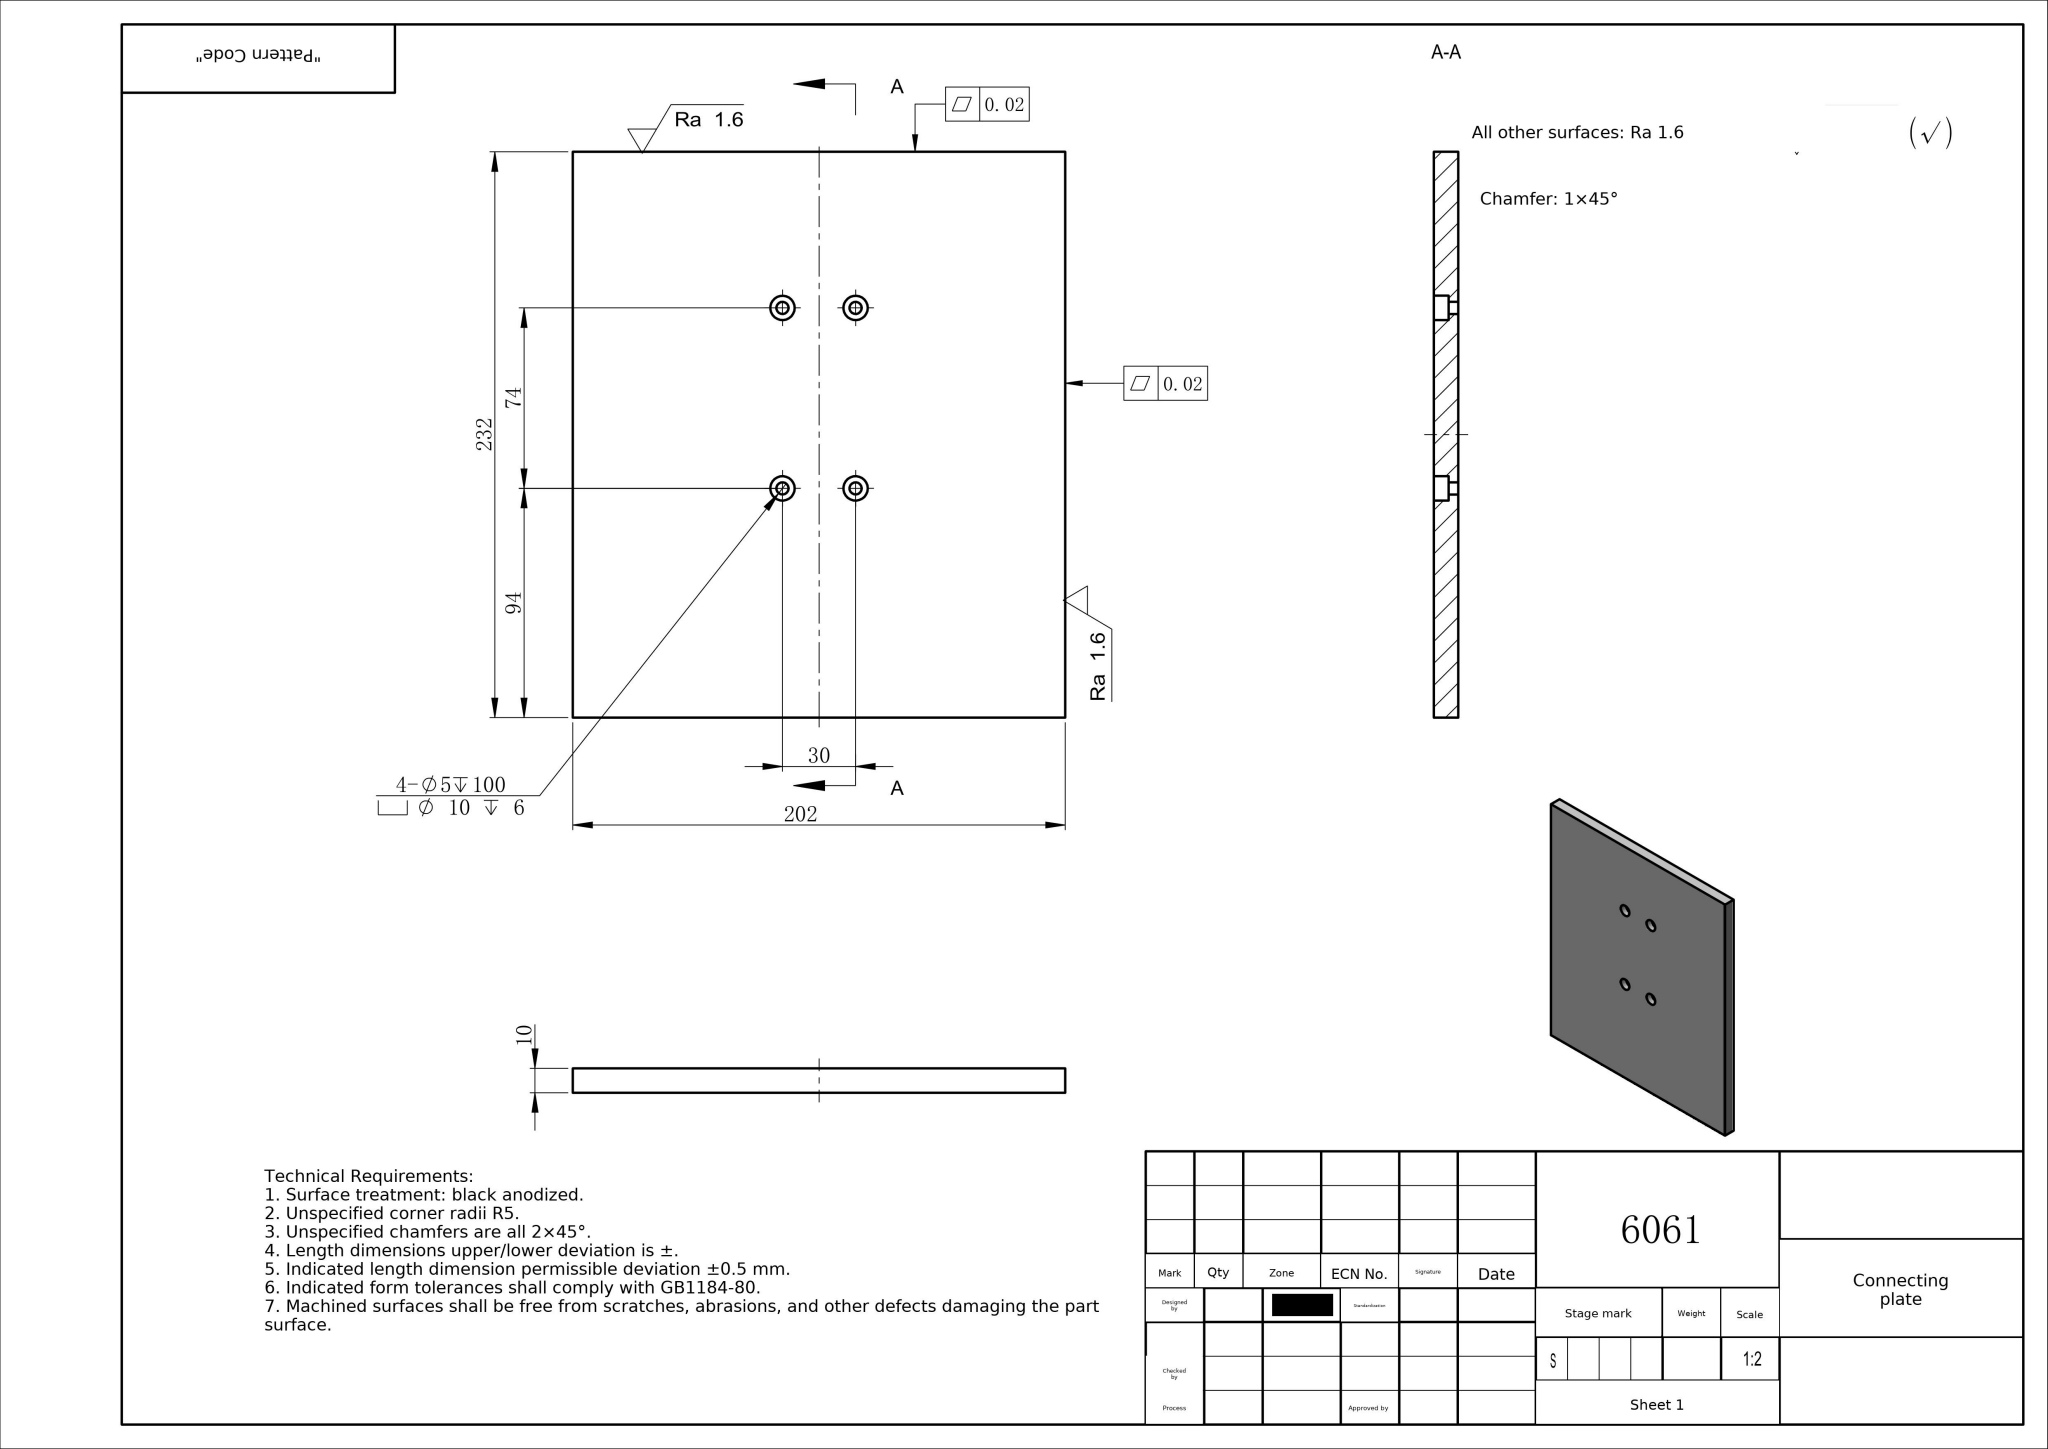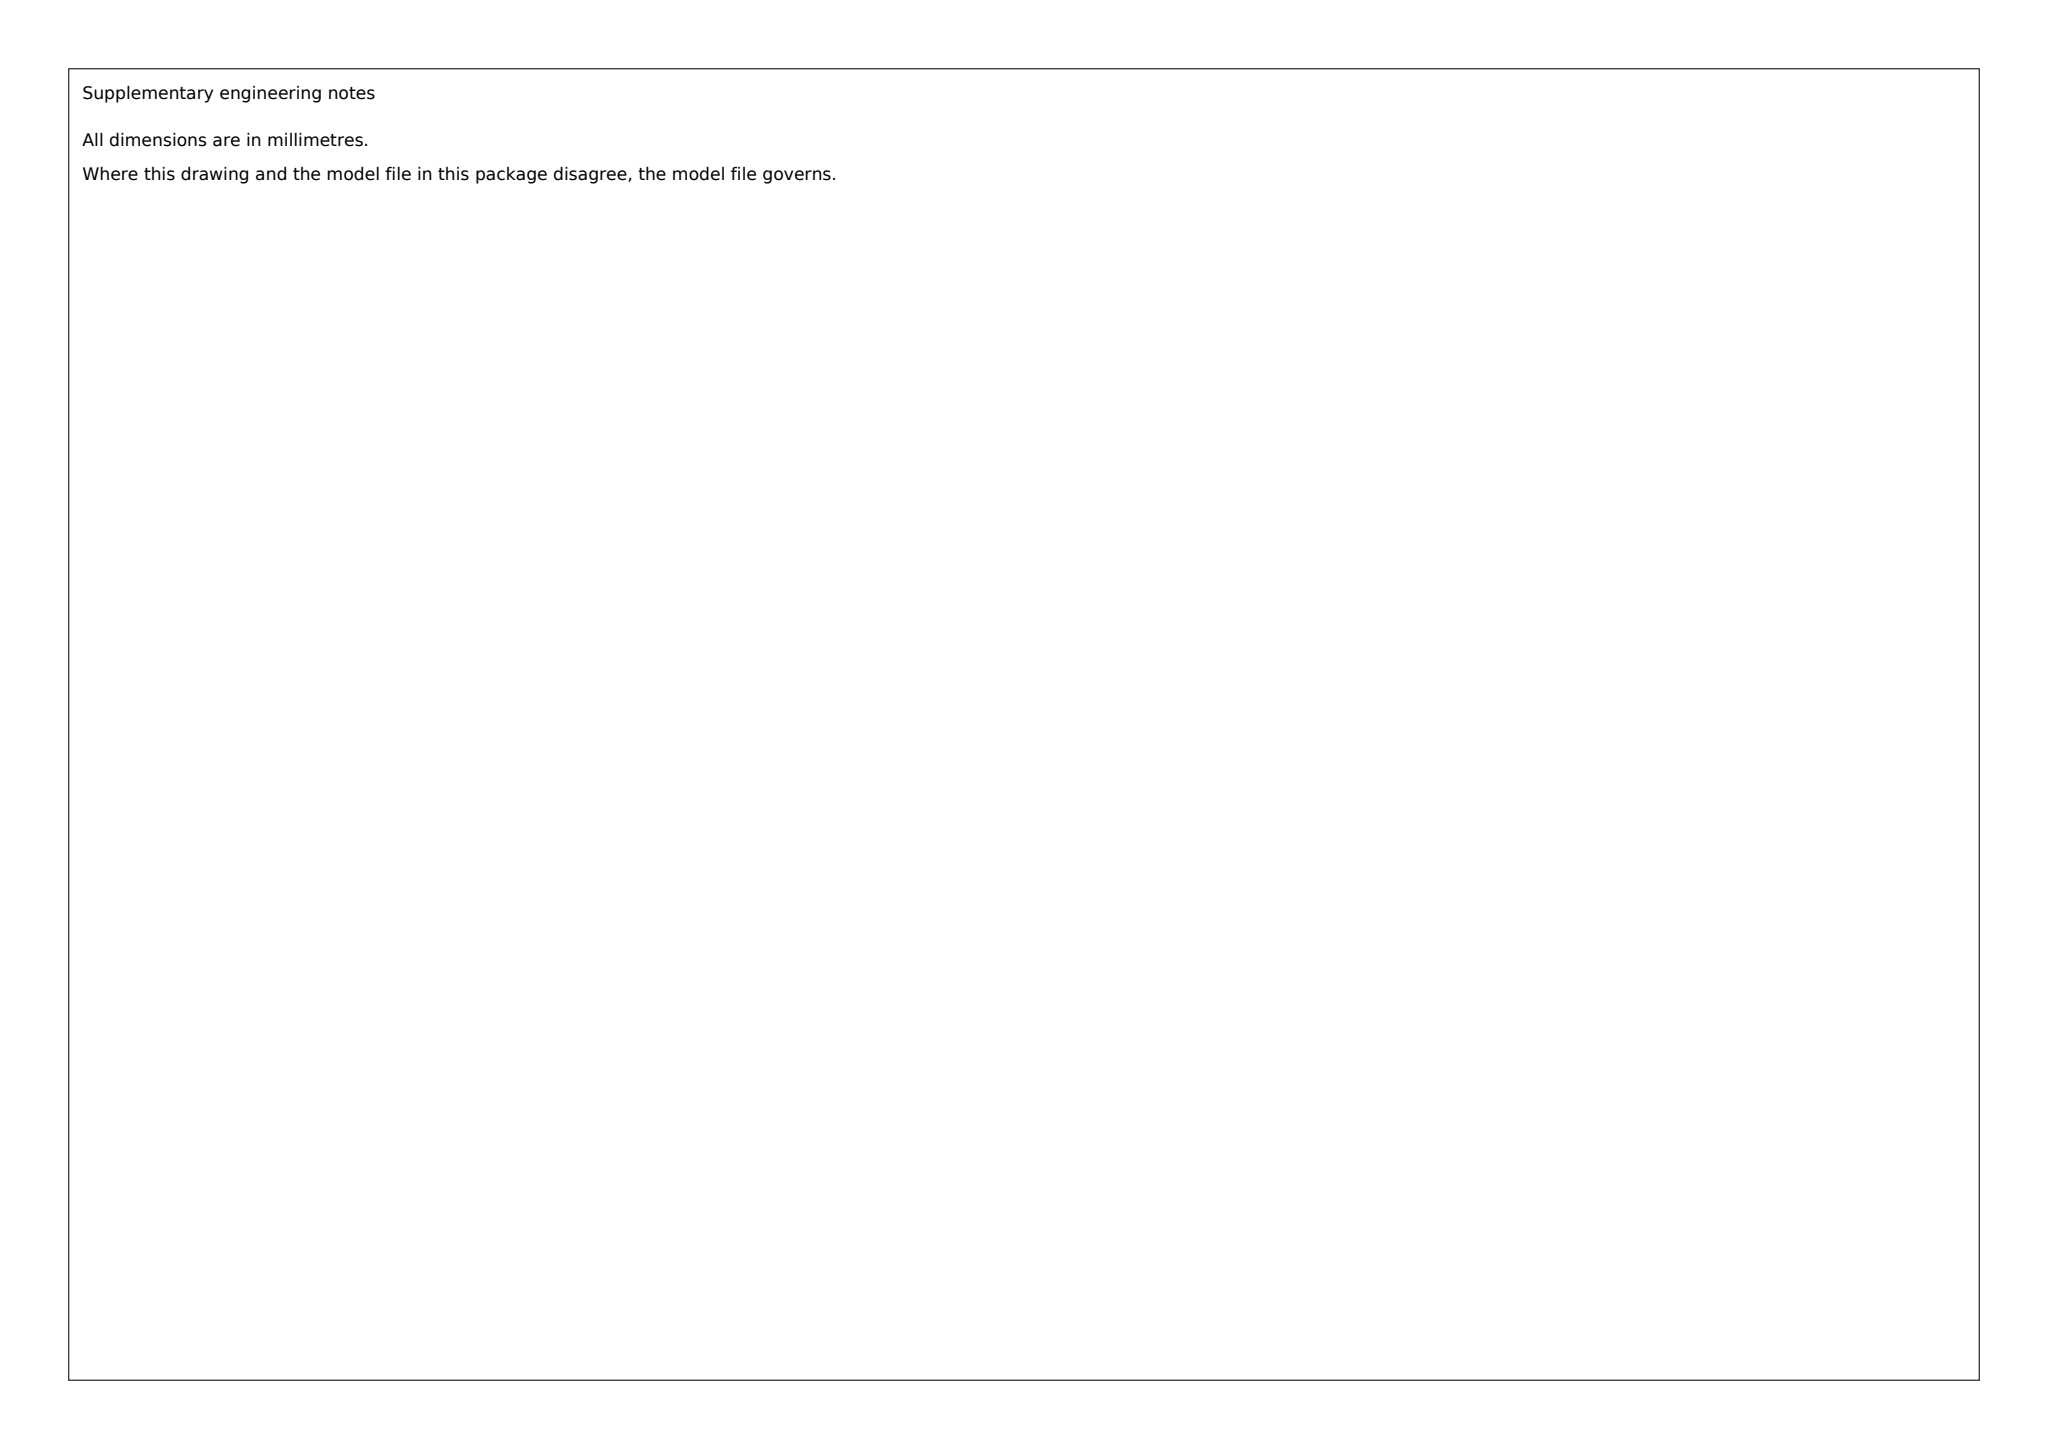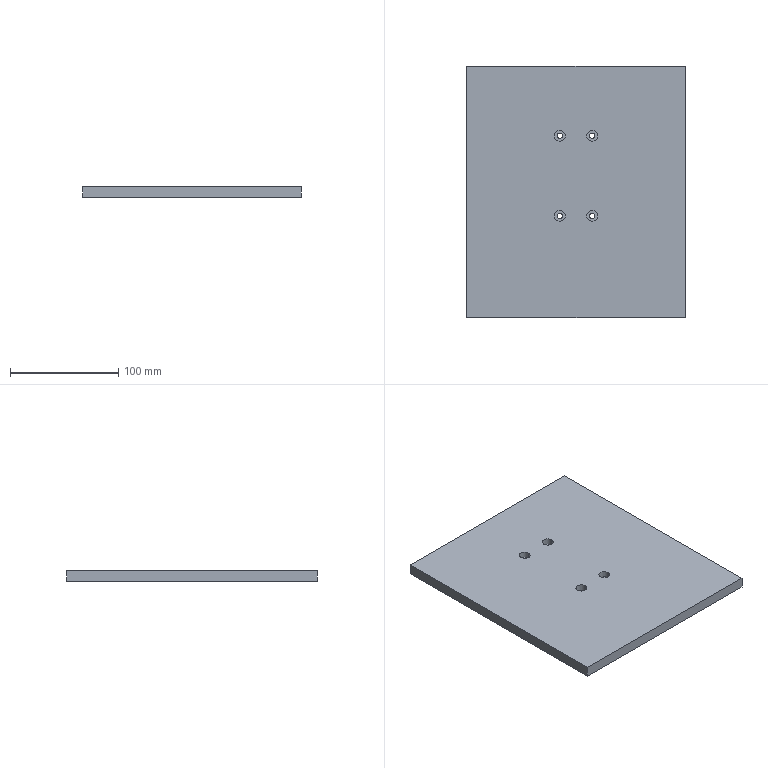Part | SolidWorks | mm | 1 solid | 26 faces | box 202 x 232 x 10 mm | volume 466441 mm3 | cylinder 16 | plane 10 | commonest cylinder face diameters 10 x8 5 x8
build123d program:
from build123d import *

# Parameters (mm, degrees)
SKETCH1_W           = 202
SKETCH1_H           = 202
BOSS_EXTRUDE1_DEPTH = 10
HOLE1_D             = 5
HOLE1_DEPTH         = 100
HOLE1_CBORE_D       = 10
HOLE1_CBORE_DEPTH   = 6
MOVE_FACE1_BY       = 30


with BuildPart() as part:
    # Sketch1 → Boss-Extrude1 (new body)
    with BuildSketch(Plane.XY):
        with Locations((-50, 0)):
            Rectangle(SKETCH1_W, SKETCH1_H)
    extrude(amount=BOSS_EXTRUDE1_DEPTH)

    # Hole1
    with Locations(Plane.XY.offset(10)):
        with Locations((-65, -37), (-65, 37), (-35, 37), (-35, -37)):
            CounterBoreHole(HOLE1_D / 2, HOLE1_CBORE_D / 2, HOLE1_CBORE_DEPTH, depth=HOLE1_DEPTH)

    # Move Face1: a face moved outward by 30.0
    extrude(part.faces().sort_by_distance((-50, -101, 5))[0], amount=MOVE_FACE1_BY, dir=(0, -1, 0))


solid = part.part
STEP:
#1=CARTESIAN_POINT('',(-70.,37.,4.));
#2=VERTEX_POINT('',#1);
#3=CARTESIAN_POINT('',(-60.,37.,4.));
#4=VERTEX_POINT('',#3);
#5=CARTESIAN_POINT('',(-65.,37.,4.));
#6=DIRECTION('',(-0.,0.,1.));
#7=DIRECTION('',(1.,0.,0.));
#8=AXIS2_PLACEMENT_3D('',#5,#6,#7);
#9=CIRCLE('',#8,5.);
#10=EDGE_CURVE('',#2,#4,#9,.T.);
#11=ORIENTED_EDGE('',*,*,#10,.F.);
#12=CARTESIAN_POINT('',(-70.,37.,10.));
#13=VERTEX_POINT('',#12);
#14=CARTESIAN_POINT('',(-70.,37.,10.));
#15=DIRECTION('',(-0.,0.,1.));
#16=VECTOR('',#15,1000.);
#17=LINE('',#14,#16);
#18=EDGE_CURVE('',#2,#13,#17,.T.);
#19=ORIENTED_EDGE('',*,*,#18,.T.);
#20=CARTESIAN_POINT('',(-60.,37.,10.));
#21=VERTEX_POINT('',#20);
#22=CARTESIAN_POINT('',(-65.,37.,10.));
#23=DIRECTION('',(-0.,0.,1.));
#24=DIRECTION('',(1.,0.,0.));
#25=AXIS2_PLACEMENT_3D('',#22,#23,#24);
#26=CIRCLE('',#25,5.);
#27=EDGE_CURVE('',#13,#21,#26,.T.);
#28=ORIENTED_EDGE('',*,*,#27,.T.);
#29=CARTESIAN_POINT('',(-60.,37.,10.));
#30=DIRECTION('',(-0.,0.,1.));
#31=VECTOR('',#30,1000.);
#32=LINE('',#29,#31);
#33=EDGE_CURVE('',#4,#21,#32,.T.);
#34=ORIENTED_EDGE('',*,*,#33,.F.);
#35=EDGE_LOOP('',(#11,#19,#28,#34));
#36=FACE_OUTER_BOUND('',#35,.T.);
#37=CARTESIAN_POINT('',(-65.,37.,10.));
#38=DIRECTION('',(-0.,0.,1.));
#39=DIRECTION('',(1.,0.,0.));
#40=AXIS2_PLACEMENT_3D('',#37,#38,#39);
#41=CYLINDRICAL_SURFACE('',#40,5.);
#42=ADVANCED_FACE('',(#36),#41,.F.);
#43=CARTESIAN_POINT('',(-67.5,37.,0.));
#44=VERTEX_POINT('',#43);
#45=CARTESIAN_POINT('',(-62.5,37.,0.));
#46=VERTEX_POINT('',#45);
#47=CARTESIAN_POINT('',(-65.,37.,0.));
#48=DIRECTION('',(-0.,0.,1.));
#49=DIRECTION('',(1.,0.,0.));
#50=AXIS2_PLACEMENT_3D('',#47,#48,#49);
#51=CIRCLE('',#50,2.5);
#52=EDGE_CURVE('',#44,#46,#51,.T.);
#53=ORIENTED_EDGE('',*,*,#52,.F.);
#54=CARTESIAN_POINT('',(-67.5,37.,4.));
#55=VERTEX_POINT('',#54);
#56=CARTESIAN_POINT('',(-67.5,37.,10.));
#57=DIRECTION('',(-0.,0.,1.));
#58=VECTOR('',#57,1000.);
#59=LINE('',#56,#58);
#60=EDGE_CURVE('',#44,#55,#59,.T.);
#61=ORIENTED_EDGE('',*,*,#60,.T.);
#62=CARTESIAN_POINT('',(-62.5,37.,4.));
#63=VERTEX_POINT('',#62);
#64=CARTESIAN_POINT('',(-65.,37.,4.));
#65=DIRECTION('',(-0.,0.,1.));
#66=DIRECTION('',(1.,0.,0.));
#67=AXIS2_PLACEMENT_3D('',#64,#65,#66);
#68=CIRCLE('',#67,2.5);
#69=EDGE_CURVE('',#55,#63,#68,.T.);
#70=ORIENTED_EDGE('',*,*,#69,.T.);
#71=CARTESIAN_POINT('',(-62.5,37.,10.));
#72=DIRECTION('',(-0.,0.,1.));
#73=VECTOR('',#72,1000.);
#74=LINE('',#71,#73);
#75=EDGE_CURVE('',#46,#63,#74,.T.);
#76=ORIENTED_EDGE('',*,*,#75,.F.);
#77=EDGE_LOOP('',(#53,#61,#70,#76));
#78=FACE_OUTER_BOUND('',#77,.T.);
#79=CARTESIAN_POINT('',(-65.,37.,10.));
#80=DIRECTION('',(-0.,0.,1.));
#81=DIRECTION('',(1.,0.,0.));
#82=AXIS2_PLACEMENT_3D('',#79,#80,#81);
#83=CYLINDRICAL_SURFACE('',#82,2.5);
#84=ADVANCED_FACE('',(#78),#83,.F.);
#85=CARTESIAN_POINT('',(-40.,37.,4.));
#86=VERTEX_POINT('',#85);
#87=CARTESIAN_POINT('',(-30.,37.,4.));
#88=VERTEX_POINT('',#87);
#89=CARTESIAN_POINT('',(-35.,37.,4.));
#90=DIRECTION('',(-0.,0.,1.));
#91=DIRECTION('',(1.,0.,0.));
#92=AXIS2_PLACEMENT_3D('',#89,#90,#91);
#93=CIRCLE('',#92,5.);
#94=EDGE_CURVE('',#86,#88,#93,.T.);
#95=ORIENTED_EDGE('',*,*,#94,.F.);
#96=CARTESIAN_POINT('',(-40.,37.,10.));
#97=VERTEX_POINT('',#96);
#98=CARTESIAN_POINT('',(-40.,37.,10.));
#99=DIRECTION('',(-0.,0.,1.));
#100=VECTOR('',#99,1000.);
#101=LINE('',#98,#100);
#102=EDGE_CURVE('',#86,#97,#101,.T.);
#103=ORIENTED_EDGE('',*,*,#102,.T.);
#104=CARTESIAN_POINT('',(-30.,37.,10.));
#105=VERTEX_POINT('',#104);
#106=CARTESIAN_POINT('',(-35.,37.,10.));
#107=DIRECTION('',(-0.,0.,1.));
#108=DIRECTION('',(1.,0.,0.));
#109=AXIS2_PLACEMENT_3D('',#106,#107,#108);
#110=CIRCLE('',#109,5.);
#111=EDGE_CURVE('',#97,#105,#110,.T.);
#112=ORIENTED_EDGE('',*,*,#111,.T.);
#113=CARTESIAN_POINT('',(-30.,37.,10.));
#114=DIRECTION('',(-0.,0.,1.));
#115=VECTOR('',#114,1000.);
#116=LINE('',#113,#115);
#117=EDGE_CURVE('',#88,#105,#116,.T.);
#118=ORIENTED_EDGE('',*,*,#117,.F.);
#119=EDGE_LOOP('',(#95,#103,#112,#118));
#120=FACE_OUTER_BOUND('',#119,.T.);
#121=CARTESIAN_POINT('',(-35.,37.,10.));
#122=DIRECTION('',(-0.,0.,1.));
#123=DIRECTION('',(1.,0.,0.));
#124=AXIS2_PLACEMENT_3D('',#121,#122,#123);
#125=CYLINDRICAL_SURFACE('',#124,5.);
#126=ADVANCED_FACE('',(#120),#125,.F.);
#127=CARTESIAN_POINT('',(-37.5,37.,0.));
#128=VERTEX_POINT('',#127);
#129=CARTESIAN_POINT('',(-32.5,37.,0.));
#130=VERTEX_POINT('',#129);
#131=CARTESIAN_POINT('',(-35.,37.,0.));
#132=DIRECTION('',(-0.,0.,1.));
#133=DIRECTION('',(1.,0.,0.));
#134=AXIS2_PLACEMENT_3D('',#131,#132,#133);
#135=CIRCLE('',#134,2.5);
#136=EDGE_CURVE('',#128,#130,#135,.T.);
#137=ORIENTED_EDGE('',*,*,#136,.F.);
#138=CARTESIAN_POINT('',(-37.5,37.,4.));
#139=VERTEX_POINT('',#138);
#140=CARTESIAN_POINT('',(-37.5,37.,10.));
#141=DIRECTION('',(-0.,0.,1.));
#142=VECTOR('',#141,1000.);
#143=LINE('',#140,#142);
#144=EDGE_CURVE('',#128,#139,#143,.T.);
#145=ORIENTED_EDGE('',*,*,#144,.T.);
#146=CARTESIAN_POINT('',(-32.5,37.,4.));
#147=VERTEX_POINT('',#146);
#148=CARTESIAN_POINT('',(-35.,37.,4.));
#149=DIRECTION('',(-0.,0.,1.));
#150=DIRECTION('',(1.,0.,0.));
#151=AXIS2_PLACEMENT_3D('',#148,#149,#150);
#152=CIRCLE('',#151,2.5);
#153=EDGE_CURVE('',#139,#147,#152,.T.);
#154=ORIENTED_EDGE('',*,*,#153,.T.);
#155=CARTESIAN_POINT('',(-32.5,37.,10.));
#156=DIRECTION('',(-0.,0.,1.));
#157=VECTOR('',#156,1000.);
#158=LINE('',#155,#157);
#159=EDGE_CURVE('',#130,#147,#158,.T.);
#160=ORIENTED_EDGE('',*,*,#159,.F.);
#161=EDGE_LOOP('',(#137,#145,#154,#160));
#162=FACE_OUTER_BOUND('',#161,.T.);
#163=CARTESIAN_POINT('',(-35.,37.,10.));
#164=DIRECTION('',(-0.,0.,1.));
#165=DIRECTION('',(1.,0.,0.));
#166=AXIS2_PLACEMENT_3D('',#163,#164,#165);
#167=CYLINDRICAL_SURFACE('',#166,2.5);
#168=ADVANCED_FACE('',(#162),#167,.F.);
#169=CARTESIAN_POINT('',(-40.,-37.,4.));
#170=VERTEX_POINT('',#169);
#171=CARTESIAN_POINT('',(-30.,-37.,4.));
#172=VERTEX_POINT('',#171);
#173=CARTESIAN_POINT('',(-35.,-37.,4.));
#174=DIRECTION('',(-0.,0.,1.));
#175=DIRECTION('',(1.,0.,0.));
#176=AXIS2_PLACEMENT_3D('',#173,#174,#175);
#177=CIRCLE('',#176,5.);
#178=EDGE_CURVE('',#170,#172,#177,.T.);
#179=ORIENTED_EDGE('',*,*,#178,.F.);
#180=CARTESIAN_POINT('',(-40.,-37.,10.));
#181=VERTEX_POINT('',#180);
#182=CARTESIAN_POINT('',(-40.,-37.,10.));
#183=DIRECTION('',(-0.,0.,1.));
#184=VECTOR('',#183,1000.);
#185=LINE('',#182,#184);
#186=EDGE_CURVE('',#170,#181,#185,.T.);
#187=ORIENTED_EDGE('',*,*,#186,.T.);
#188=CARTESIAN_POINT('',(-30.,-37.,10.));
#189=VERTEX_POINT('',#188);
#190=CARTESIAN_POINT('',(-35.,-37.,10.));
#191=DIRECTION('',(-0.,0.,1.));
#192=DIRECTION('',(1.,0.,0.));
#193=AXIS2_PLACEMENT_3D('',#190,#191,#192);
#194=CIRCLE('',#193,5.);
#195=EDGE_CURVE('',#181,#189,#194,.T.);
#196=ORIENTED_EDGE('',*,*,#195,.T.);
#197=CARTESIAN_POINT('',(-30.,-37.,10.));
#198=DIRECTION('',(-0.,0.,1.));
#199=VECTOR('',#198,1000.);
#200=LINE('',#197,#199);
#201=EDGE_CURVE('',#172,#189,#200,.T.);
#202=ORIENTED_EDGE('',*,*,#201,.F.);
#203=EDGE_LOOP('',(#179,#187,#196,#202));
#204=FACE_OUTER_BOUND('',#203,.T.);
#205=CARTESIAN_POINT('',(-35.,-37.,10.));
#206=DIRECTION('',(-0.,0.,1.));
#207=DIRECTION('',(1.,0.,0.));
#208=AXIS2_PLACEMENT_3D('',#205,#206,#207);
#209=CYLINDRICAL_SURFACE('',#208,5.);
#210=ADVANCED_FACE('',(#204),#209,.F.);
#211=CARTESIAN_POINT('',(-37.5,-37.,-0.));
#212=VERTEX_POINT('',#211);
#213=CARTESIAN_POINT('',(-32.5,-37.,-0.));
#214=VERTEX_POINT('',#213);
#215=CARTESIAN_POINT('',(-35.,-37.,0.));
#216=DIRECTION('',(-0.,0.,1.));
#217=DIRECTION('',(1.,0.,-0.));
#218=AXIS2_PLACEMENT_3D('',#215,#216,#217);
#219=CIRCLE('',#218,2.5);
#220=EDGE_CURVE('',#212,#214,#219,.T.);
#221=ORIENTED_EDGE('',*,*,#220,.F.);
#222=CARTESIAN_POINT('',(-37.5,-37.,4.));
#223=VERTEX_POINT('',#222);
#224=CARTESIAN_POINT('',(-37.5,-37.,10.));
#225=DIRECTION('',(-0.,0.,1.));
#226=VECTOR('',#225,1000.);
#227=LINE('',#224,#226);
#228=EDGE_CURVE('',#212,#223,#227,.T.);
#229=ORIENTED_EDGE('',*,*,#228,.T.);
#230=CARTESIAN_POINT('',(-32.5,-37.,4.));
#231=VERTEX_POINT('',#230);
#232=CARTESIAN_POINT('',(-35.,-37.,4.));
#233=DIRECTION('',(-0.,0.,1.));
#234=DIRECTION('',(1.,0.,0.));
#235=AXIS2_PLACEMENT_3D('',#232,#233,#234);
#236=CIRCLE('',#235,2.5);
#237=EDGE_CURVE('',#223,#231,#236,.T.);
#238=ORIENTED_EDGE('',*,*,#237,.T.);
#239=CARTESIAN_POINT('',(-32.5,-37.,10.));
#240=DIRECTION('',(-0.,0.,1.));
#241=VECTOR('',#240,1000.);
#242=LINE('',#239,#241);
#243=EDGE_CURVE('',#214,#231,#242,.T.);
#244=ORIENTED_EDGE('',*,*,#243,.F.);
#245=EDGE_LOOP('',(#221,#229,#238,#244));
#246=FACE_OUTER_BOUND('',#245,.T.);
#247=CARTESIAN_POINT('',(-35.,-37.,10.));
#248=DIRECTION('',(-0.,0.,1.));
#249=DIRECTION('',(1.,0.,0.));
#250=AXIS2_PLACEMENT_3D('',#247,#248,#249);
#251=CYLINDRICAL_SURFACE('',#250,2.5);
#252=ADVANCED_FACE('',(#246),#251,.F.);
#253=CARTESIAN_POINT('',(-70.,-37.,4.));
#254=VERTEX_POINT('',#253);
#255=CARTESIAN_POINT('',(-60.,-37.,4.));
#256=VERTEX_POINT('',#255);
#257=CARTESIAN_POINT('',(-65.,-37.,4.));
#258=DIRECTION('',(-0.,0.,1.));
#259=DIRECTION('',(1.,0.,0.));
#260=AXIS2_PLACEMENT_3D('',#257,#258,#259);
#261=CIRCLE('',#260,5.);
#262=EDGE_CURVE('',#254,#256,#261,.T.);
#263=ORIENTED_EDGE('',*,*,#262,.F.);
#264=CARTESIAN_POINT('',(-70.,-37.,10.));
#265=VERTEX_POINT('',#264);
#266=CARTESIAN_POINT('',(-70.,-37.,10.));
#267=DIRECTION('',(-0.,0.,1.));
#268=VECTOR('',#267,1000.);
#269=LINE('',#266,#268);
#270=EDGE_CURVE('',#254,#265,#269,.T.);
#271=ORIENTED_EDGE('',*,*,#270,.T.);
#272=CARTESIAN_POINT('',(-60.,-37.,10.));
#273=VERTEX_POINT('',#272);
#274=CARTESIAN_POINT('',(-65.,-37.,10.));
#275=DIRECTION('',(-0.,0.,1.));
#276=DIRECTION('',(1.,0.,0.));
#277=AXIS2_PLACEMENT_3D('',#274,#275,#276);
#278=CIRCLE('',#277,5.);
#279=EDGE_CURVE('',#265,#273,#278,.T.);
#280=ORIENTED_EDGE('',*,*,#279,.T.);
#281=CARTESIAN_POINT('',(-60.,-37.,10.));
#282=DIRECTION('',(-0.,0.,1.));
#283=VECTOR('',#282,1000.);
#284=LINE('',#281,#283);
#285=EDGE_CURVE('',#256,#273,#284,.T.);
#286=ORIENTED_EDGE('',*,*,#285,.F.);
#287=EDGE_LOOP('',(#263,#271,#280,#286));
#288=FACE_OUTER_BOUND('',#287,.T.);
#289=CARTESIAN_POINT('',(-65.,-37.,10.));
#290=DIRECTION('',(-0.,0.,1.));
#291=DIRECTION('',(1.,0.,0.));
#292=AXIS2_PLACEMENT_3D('',#289,#290,#291);
#293=CYLINDRICAL_SURFACE('',#292,5.);
#294=ADVANCED_FACE('',(#288),#293,.F.);
#295=CARTESIAN_POINT('',(-67.5,-37.,-0.));
#296=VERTEX_POINT('',#295);
#297=CARTESIAN_POINT('',(-62.5,-37.,-0.));
#298=VERTEX_POINT('',#297);
#299=CARTESIAN_POINT('',(-65.,-37.,0.));
#300=DIRECTION('',(-0.,0.,1.));
#301=DIRECTION('',(1.,0.,-0.));
#302=AXIS2_PLACEMENT_3D('',#299,#300,#301);
#303=CIRCLE('',#302,2.5);
#304=EDGE_CURVE('',#296,#298,#303,.T.);
#305=ORIENTED_EDGE('',*,*,#304,.F.);
#306=CARTESIAN_POINT('',(-67.5,-37.,4.));
#307=VERTEX_POINT('',#306);
#308=CARTESIAN_POINT('',(-67.5,-37.,10.));
#309=DIRECTION('',(-0.,0.,1.));
#310=VECTOR('',#309,1000.);
#311=LINE('',#308,#310);
#312=EDGE_CURVE('',#296,#307,#311,.T.);
#313=ORIENTED_EDGE('',*,*,#312,.T.);
#314=CARTESIAN_POINT('',(-62.5,-37.,4.));
#315=VERTEX_POINT('',#314);
#316=CARTESIAN_POINT('',(-65.,-37.,4.));
#317=DIRECTION('',(-0.,0.,1.));
#318=DIRECTION('',(1.,0.,0.));
#319=AXIS2_PLACEMENT_3D('',#316,#317,#318);
#320=CIRCLE('',#319,2.5);
#321=EDGE_CURVE('',#307,#315,#320,.T.);
#322=ORIENTED_EDGE('',*,*,#321,.T.);
#323=CARTESIAN_POINT('',(-62.5,-37.,10.));
#324=DIRECTION('',(-0.,0.,1.));
#325=VECTOR('',#324,1000.);
#326=LINE('',#323,#325);
#327=EDGE_CURVE('',#298,#315,#326,.T.);
#328=ORIENTED_EDGE('',*,*,#327,.F.);
#329=EDGE_LOOP('',(#305,#313,#322,#328));
#330=FACE_OUTER_BOUND('',#329,.T.);
#331=CARTESIAN_POINT('',(-65.,-37.,10.));
#332=DIRECTION('',(-0.,0.,1.));
#333=DIRECTION('',(1.,0.,0.));
#334=AXIS2_PLACEMENT_3D('',#331,#332,#333);
#335=CYLINDRICAL_SURFACE('',#334,2.5);
#336=ADVANCED_FACE('',(#330),#335,.F.);
#337=CARTESIAN_POINT('',(51.,-131.,0.));
#338=VERTEX_POINT('',#337);
#339=CARTESIAN_POINT('',(51.,101.,0.));
#340=VERTEX_POINT('',#339);
#341=CARTESIAN_POINT('',(51.,101.,0.));
#342=DIRECTION('',(-0.,1.,0.));
#343=VECTOR('',#342,1000.);
#344=LINE('',#341,#343);
#345=EDGE_CURVE('',#338,#340,#344,.T.);
#346=ORIENTED_EDGE('',*,*,#345,.T.);
#347=CARTESIAN_POINT('',(51.,101.,10.));
#348=VERTEX_POINT('',#347);
#349=CARTESIAN_POINT('',(51.,101.,10.));
#350=DIRECTION('',(0.,-0.,-1.));
#351=VECTOR('',#350,1000.);
#352=LINE('',#349,#351);
#353=EDGE_CURVE('',#348,#340,#352,.T.);
#354=ORIENTED_EDGE('',*,*,#353,.F.);
#355=CARTESIAN_POINT('',(51.,-131.,10.));
#356=VERTEX_POINT('',#355);
#357=CARTESIAN_POINT('',(51.,101.,10.));
#358=DIRECTION('',(-0.,1.,0.));
#359=VECTOR('',#358,1000.);
#360=LINE('',#357,#359);
#361=EDGE_CURVE('',#356,#348,#360,.T.);
#362=ORIENTED_EDGE('',*,*,#361,.F.);
#363=CARTESIAN_POINT('',(51.,-131.,10.));
#364=DIRECTION('',(0.,-0.,-1.));
#365=VECTOR('',#364,1000.);
#366=LINE('',#363,#365);
#367=EDGE_CURVE('',#356,#338,#366,.T.);
#368=ORIENTED_EDGE('',*,*,#367,.T.);
#369=EDGE_LOOP('',(#346,#354,#362,#368));
#370=FACE_OUTER_BOUND('',#369,.T.);
#371=CARTESIAN_POINT('',(51.,101.,10.));
#372=DIRECTION('',(-1.,-0.,0.));
#373=DIRECTION('',(0.,-1.,-0.));
#374=AXIS2_PLACEMENT_3D('',#371,#372,#373);
#375=PLANE('',#374);
#376=ADVANCED_FACE('',(#370),#375,.F.);
#377=CARTESIAN_POINT('',(-151.,101.,0.));
#378=VERTEX_POINT('',#377);
#379=CARTESIAN_POINT('',(-151.,101.,0.));
#380=DIRECTION('',(-1.,-0.,0.));
#381=VECTOR('',#380,1000.);
#382=LINE('',#379,#381);
#383=EDGE_CURVE('',#340,#378,#382,.T.);
#384=ORIENTED_EDGE('',*,*,#383,.T.);
#385=CARTESIAN_POINT('',(-151.,101.,10.));
#386=VERTEX_POINT('',#385);
#387=CARTESIAN_POINT('',(-151.,101.,10.));
#388=DIRECTION('',(0.,-0.,-1.));
#389=VECTOR('',#388,1000.);
#390=LINE('',#387,#389);
#391=EDGE_CURVE('',#386,#378,#390,.T.);
#392=ORIENTED_EDGE('',*,*,#391,.F.);
#393=CARTESIAN_POINT('',(-151.,101.,10.));
#394=DIRECTION('',(-1.,-0.,0.));
#395=VECTOR('',#394,1000.);
#396=LINE('',#393,#395);
#397=EDGE_CURVE('',#348,#386,#396,.T.);
#398=ORIENTED_EDGE('',*,*,#397,.F.);
#399=ORIENTED_EDGE('',*,*,#353,.T.);
#400=EDGE_LOOP('',(#384,#392,#398,#399));
#401=FACE_OUTER_BOUND('',#400,.T.);
#402=CARTESIAN_POINT('',(-151.,101.,10.));
#403=DIRECTION('',(-0.,-1.,0.));
#404=DIRECTION('',(0.,-0.,-1.));
#405=AXIS2_PLACEMENT_3D('',#402,#403,#404);
#406=PLANE('',#405);
#407=ADVANCED_FACE('',(#401),#406,.F.);
#408=CARTESIAN_POINT('',(-151.,-131.,0.));
#409=VERTEX_POINT('',#408);
#410=CARTESIAN_POINT('',(-151.,101.,0.));
#411=DIRECTION('',(-0.,-1.,-0.));
#412=VECTOR('',#411,1000.);
#413=LINE('',#410,#412);
#414=EDGE_CURVE('',#378,#409,#413,.T.);
#415=ORIENTED_EDGE('',*,*,#414,.T.);
#416=CARTESIAN_POINT('',(-151.,-131.,10.));
#417=VERTEX_POINT('',#416);
#418=CARTESIAN_POINT('',(-151.,-131.,10.));
#419=DIRECTION('',(0.,-0.,-1.));
#420=VECTOR('',#419,1000.);
#421=LINE('',#418,#420);
#422=EDGE_CURVE('',#417,#409,#421,.T.);
#423=ORIENTED_EDGE('',*,*,#422,.F.);
#424=CARTESIAN_POINT('',(-151.,101.,10.));
#425=DIRECTION('',(-0.,-1.,-0.));
#426=VECTOR('',#425,1000.);
#427=LINE('',#424,#426);
#428=EDGE_CURVE('',#386,#417,#427,.T.);
#429=ORIENTED_EDGE('',*,*,#428,.F.);
#430=ORIENTED_EDGE('',*,*,#391,.T.);
#431=EDGE_LOOP('',(#415,#423,#429,#430));
#432=FACE_OUTER_BOUND('',#431,.T.);
#433=CARTESIAN_POINT('',(-151.,101.,10.));
#434=DIRECTION('',(1.,0.,0.));
#435=DIRECTION('',(0.,-0.,-1.));
#436=AXIS2_PLACEMENT_3D('',#433,#434,#435);
#437=PLANE('',#436);
#438=ADVANCED_FACE('',(#432),#437,.F.);
#439=CARTESIAN_POINT('',(-151.,-131.,0.));
#440=DIRECTION('',(1.,0.,-0.));
#441=VECTOR('',#440,1000.);
#442=LINE('',#439,#441);
#443=EDGE_CURVE('',#409,#338,#442,.T.);
#444=ORIENTED_EDGE('',*,*,#443,.T.);
#445=ORIENTED_EDGE('',*,*,#367,.F.);
#446=CARTESIAN_POINT('',(-151.,-131.,10.));
#447=DIRECTION('',(1.,0.,-0.));
#448=VECTOR('',#447,1000.);
#449=LINE('',#446,#448);
#450=EDGE_CURVE('',#417,#356,#449,.T.);
#451=ORIENTED_EDGE('',*,*,#450,.F.);
#452=ORIENTED_EDGE('',*,*,#422,.T.);
#453=EDGE_LOOP('',(#444,#445,#451,#452));
#454=FACE_OUTER_BOUND('',#453,.T.);
#455=CARTESIAN_POINT('',(-151.,-131.,10.));
#456=DIRECTION('',(0.,1.,-0.));
#457=DIRECTION('',(-0.,0.,1.));
#458=AXIS2_PLACEMENT_3D('',#455,#456,#457);
#459=PLANE('',#458);
#460=ADVANCED_FACE('',(#454),#459,.F.);
#461=CARTESIAN_POINT('',(-65.,37.,10.));
#462=DIRECTION('',(-0.,0.,1.));
#463=DIRECTION('',(1.,0.,0.));
#464=AXIS2_PLACEMENT_3D('',#461,#462,#463);
#465=CIRCLE('',#464,5.);
#466=EDGE_CURVE('',#21,#13,#465,.T.);
#467=ORIENTED_EDGE('',*,*,#466,.F.);
#468=ORIENTED_EDGE('',*,*,#27,.F.);
#469=EDGE_LOOP('',(#467,#468));
#470=FACE_BOUND('',#469,.T.);
#471=CARTESIAN_POINT('',(-35.,37.,10.));
#472=DIRECTION('',(-0.,0.,1.));
#473=DIRECTION('',(1.,0.,0.));
#474=AXIS2_PLACEMENT_3D('',#471,#472,#473);
#475=CIRCLE('',#474,5.);
#476=EDGE_CURVE('',#105,#97,#475,.T.);
#477=ORIENTED_EDGE('',*,*,#476,.F.);
#478=ORIENTED_EDGE('',*,*,#111,.F.);
#479=EDGE_LOOP('',(#477,#478));
#480=FACE_BOUND('',#479,.T.);
#481=CARTESIAN_POINT('',(-35.,-37.,10.));
#482=DIRECTION('',(-0.,0.,1.));
#483=DIRECTION('',(1.,0.,0.));
#484=AXIS2_PLACEMENT_3D('',#481,#482,#483);
#485=CIRCLE('',#484,5.);
#486=EDGE_CURVE('',#189,#181,#485,.T.);
#487=ORIENTED_EDGE('',*,*,#486,.F.);
#488=ORIENTED_EDGE('',*,*,#195,.F.);
#489=EDGE_LOOP('',(#487,#488));
#490=FACE_BOUND('',#489,.T.);
#491=CARTESIAN_POINT('',(-65.,-37.,10.));
#492=DIRECTION('',(-0.,0.,1.));
#493=DIRECTION('',(1.,0.,0.));
#494=AXIS2_PLACEMENT_3D('',#491,#492,#493);
#495=CIRCLE('',#494,5.);
#496=EDGE_CURVE('',#273,#265,#495,.T.);
#497=ORIENTED_EDGE('',*,*,#496,.F.);
#498=ORIENTED_EDGE('',*,*,#279,.F.);
#499=EDGE_LOOP('',(#497,#498));
#500=FACE_BOUND('',#499,.T.);
#501=ORIENTED_EDGE('',*,*,#361,.T.);
#502=ORIENTED_EDGE('',*,*,#397,.T.);
#503=ORIENTED_EDGE('',*,*,#428,.T.);
#504=ORIENTED_EDGE('',*,*,#450,.T.);
#505=EDGE_LOOP('',(#501,#502,#503,#504));
#506=FACE_OUTER_BOUND('',#505,.T.);
#507=CARTESIAN_POINT('',(0.,0.,10.));
#508=DIRECTION('',(0.,0.,1.));
#509=DIRECTION('',(1.,0.,-0.));
#510=AXIS2_PLACEMENT_3D('',#507,#508,#509);
#511=PLANE('',#510);
#512=ADVANCED_FACE('',(#470,#480,#490,#500,#506),#511,.T.);
#513=CARTESIAN_POINT('',(-65.,37.,0.));
#514=DIRECTION('',(-0.,0.,1.));
#515=DIRECTION('',(1.,0.,0.));
#516=AXIS2_PLACEMENT_3D('',#513,#514,#515);
#517=CIRCLE('',#516,2.5);
#518=EDGE_CURVE('',#46,#44,#517,.T.);
#519=ORIENTED_EDGE('',*,*,#518,.T.);
#520=ORIENTED_EDGE('',*,*,#52,.T.);
#521=EDGE_LOOP('',(#519,#520));
#522=FACE_BOUND('',#521,.T.);
#523=CARTESIAN_POINT('',(-35.,37.,0.));
#524=DIRECTION('',(-0.,0.,1.));
#525=DIRECTION('',(1.,0.,0.));
#526=AXIS2_PLACEMENT_3D('',#523,#524,#525);
#527=CIRCLE('',#526,2.5);
#528=EDGE_CURVE('',#130,#128,#527,.T.);
#529=ORIENTED_EDGE('',*,*,#528,.T.);
#530=ORIENTED_EDGE('',*,*,#136,.T.);
#531=EDGE_LOOP('',(#529,#530));
#532=FACE_BOUND('',#531,.T.);
#533=CARTESIAN_POINT('',(-35.,-37.,0.));
#534=DIRECTION('',(-0.,0.,1.));
#535=DIRECTION('',(1.,0.,-0.));
#536=AXIS2_PLACEMENT_3D('',#533,#534,#535);
#537=CIRCLE('',#536,2.5);
#538=EDGE_CURVE('',#214,#212,#537,.T.);
#539=ORIENTED_EDGE('',*,*,#538,.T.);
#540=ORIENTED_EDGE('',*,*,#220,.T.);
#541=EDGE_LOOP('',(#539,#540));
#542=FACE_BOUND('',#541,.T.);
#543=CARTESIAN_POINT('',(-65.,-37.,0.));
#544=DIRECTION('',(-0.,0.,1.));
#545=DIRECTION('',(1.,0.,-0.));
#546=AXIS2_PLACEMENT_3D('',#543,#544,#545);
#547=CIRCLE('',#546,2.5);
#548=EDGE_CURVE('',#298,#296,#547,.T.);
#549=ORIENTED_EDGE('',*,*,#548,.T.);
#550=ORIENTED_EDGE('',*,*,#304,.T.);
#551=EDGE_LOOP('',(#549,#550));
#552=FACE_BOUND('',#551,.T.);
#553=ORIENTED_EDGE('',*,*,#345,.F.);
#554=ORIENTED_EDGE('',*,*,#443,.F.);
#555=ORIENTED_EDGE('',*,*,#414,.F.);
#556=ORIENTED_EDGE('',*,*,#383,.F.);
#557=EDGE_LOOP('',(#553,#554,#555,#556));
#558=FACE_OUTER_BOUND('',#557,.T.);
#559=CARTESIAN_POINT('',(0.,0.,0.));
#560=DIRECTION('',(0.,0.,1.));
#561=DIRECTION('',(1.,0.,-0.));
#562=AXIS2_PLACEMENT_3D('',#559,#560,#561);
#563=PLANE('',#562);
#564=ADVANCED_FACE('',(#522,#532,#542,#552,#558),#563,.F.);
#565=ORIENTED_EDGE('',*,*,#312,.F.);
#566=ORIENTED_EDGE('',*,*,#548,.F.);
#567=ORIENTED_EDGE('',*,*,#327,.T.);
#568=CARTESIAN_POINT('',(-65.,-37.,4.));
#569=DIRECTION('',(-0.,0.,1.));
#570=DIRECTION('',(1.,0.,0.));
#571=AXIS2_PLACEMENT_3D('',#568,#569,#570);
#572=CIRCLE('',#571,2.5);
#573=EDGE_CURVE('',#315,#307,#572,.T.);
#574=ORIENTED_EDGE('',*,*,#573,.T.);
#575=EDGE_LOOP('',(#565,#566,#567,#574));
#576=FACE_OUTER_BOUND('',#575,.T.);
#577=CARTESIAN_POINT('',(-65.,-37.,10.));
#578=DIRECTION('',(-0.,0.,1.));
#579=DIRECTION('',(1.,0.,0.));
#580=AXIS2_PLACEMENT_3D('',#577,#578,#579);
#581=CYLINDRICAL_SURFACE('',#580,2.5);
#582=ADVANCED_FACE('',(#576),#581,.F.);
#583=ORIENTED_EDGE('',*,*,#573,.F.);
#584=ORIENTED_EDGE('',*,*,#321,.F.);
#585=EDGE_LOOP('',(#583,#584));
#586=FACE_BOUND('',#585,.T.);
#587=CARTESIAN_POINT('',(-65.,-37.,4.));
#588=DIRECTION('',(-0.,0.,1.));
#589=DIRECTION('',(1.,0.,0.));
#590=AXIS2_PLACEMENT_3D('',#587,#588,#589);
#591=CIRCLE('',#590,5.);
#592=EDGE_CURVE('',#256,#254,#591,.T.);
#593=ORIENTED_EDGE('',*,*,#592,.T.);
#594=ORIENTED_EDGE('',*,*,#262,.T.);
#595=EDGE_LOOP('',(#593,#594));
#596=FACE_OUTER_BOUND('',#595,.T.);
#597=CARTESIAN_POINT('',(-62.5,-37.,4.));
#598=DIRECTION('',(-0.,-0.,-1.));
#599=DIRECTION('',(-1.,-0.,0.));
#600=AXIS2_PLACEMENT_3D('',#597,#598,#599);
#601=PLANE('',#600);
#602=ADVANCED_FACE('',(#586,#596),#601,.F.);
#603=ORIENTED_EDGE('',*,*,#270,.F.);
#604=ORIENTED_EDGE('',*,*,#592,.F.);
#605=ORIENTED_EDGE('',*,*,#285,.T.);
#606=ORIENTED_EDGE('',*,*,#496,.T.);
#607=EDGE_LOOP('',(#603,#604,#605,#606));
#608=FACE_OUTER_BOUND('',#607,.T.);
#609=CARTESIAN_POINT('',(-65.,-37.,10.));
#610=DIRECTION('',(-0.,0.,1.));
#611=DIRECTION('',(1.,0.,0.));
#612=AXIS2_PLACEMENT_3D('',#609,#610,#611);
#613=CYLINDRICAL_SURFACE('',#612,5.);
#614=ADVANCED_FACE('',(#608),#613,.F.);
#615=ORIENTED_EDGE('',*,*,#228,.F.);
#616=ORIENTED_EDGE('',*,*,#538,.F.);
#617=ORIENTED_EDGE('',*,*,#243,.T.);
#618=CARTESIAN_POINT('',(-35.,-37.,4.));
#619=DIRECTION('',(-0.,0.,1.));
#620=DIRECTION('',(1.,0.,0.));
#621=AXIS2_PLACEMENT_3D('',#618,#619,#620);
#622=CIRCLE('',#621,2.5);
#623=EDGE_CURVE('',#231,#223,#622,.T.);
#624=ORIENTED_EDGE('',*,*,#623,.T.);
#625=EDGE_LOOP('',(#615,#616,#617,#624));
#626=FACE_OUTER_BOUND('',#625,.T.);
#627=CARTESIAN_POINT('',(-35.,-37.,10.));
#628=DIRECTION('',(-0.,0.,1.));
#629=DIRECTION('',(1.,0.,0.));
#630=AXIS2_PLACEMENT_3D('',#627,#628,#629);
#631=CYLINDRICAL_SURFACE('',#630,2.5);
#632=ADVANCED_FACE('',(#626),#631,.F.);
#633=ORIENTED_EDGE('',*,*,#623,.F.);
#634=ORIENTED_EDGE('',*,*,#237,.F.);
#635=EDGE_LOOP('',(#633,#634));
#636=FACE_BOUND('',#635,.T.);
#637=CARTESIAN_POINT('',(-35.,-37.,4.));
#638=DIRECTION('',(-0.,0.,1.));
#639=DIRECTION('',(1.,0.,0.));
#640=AXIS2_PLACEMENT_3D('',#637,#638,#639);
#641=CIRCLE('',#640,5.);
#642=EDGE_CURVE('',#172,#170,#641,.T.);
#643=ORIENTED_EDGE('',*,*,#642,.T.);
#644=ORIENTED_EDGE('',*,*,#178,.T.);
#645=EDGE_LOOP('',(#643,#644));
#646=FACE_OUTER_BOUND('',#645,.T.);
#647=CARTESIAN_POINT('',(-32.5,-37.,4.));
#648=DIRECTION('',(-0.,-0.,-1.));
#649=DIRECTION('',(-1.,-0.,0.));
#650=AXIS2_PLACEMENT_3D('',#647,#648,#649);
#651=PLANE('',#650);
#652=ADVANCED_FACE('',(#636,#646),#651,.F.);
#653=ORIENTED_EDGE('',*,*,#186,.F.);
#654=ORIENTED_EDGE('',*,*,#642,.F.);
#655=ORIENTED_EDGE('',*,*,#201,.T.);
#656=ORIENTED_EDGE('',*,*,#486,.T.);
#657=EDGE_LOOP('',(#653,#654,#655,#656));
#658=FACE_OUTER_BOUND('',#657,.T.);
#659=CARTESIAN_POINT('',(-35.,-37.,10.));
#660=DIRECTION('',(-0.,0.,1.));
#661=DIRECTION('',(1.,0.,0.));
#662=AXIS2_PLACEMENT_3D('',#659,#660,#661);
#663=CYLINDRICAL_SURFACE('',#662,5.);
#664=ADVANCED_FACE('',(#658),#663,.F.);
#665=ORIENTED_EDGE('',*,*,#144,.F.);
#666=ORIENTED_EDGE('',*,*,#528,.F.);
#667=ORIENTED_EDGE('',*,*,#159,.T.);
#668=CARTESIAN_POINT('',(-35.,37.,4.));
#669=DIRECTION('',(-0.,0.,1.));
#670=DIRECTION('',(1.,0.,0.));
#671=AXIS2_PLACEMENT_3D('',#668,#669,#670);
#672=CIRCLE('',#671,2.5);
#673=EDGE_CURVE('',#147,#139,#672,.T.);
#674=ORIENTED_EDGE('',*,*,#673,.T.);
#675=EDGE_LOOP('',(#665,#666,#667,#674));
#676=FACE_OUTER_BOUND('',#675,.T.);
#677=CARTESIAN_POINT('',(-35.,37.,10.));
#678=DIRECTION('',(-0.,0.,1.));
#679=DIRECTION('',(1.,0.,0.));
#680=AXIS2_PLACEMENT_3D('',#677,#678,#679);
#681=CYLINDRICAL_SURFACE('',#680,2.5);
#682=ADVANCED_FACE('',(#676),#681,.F.);
#683=ORIENTED_EDGE('',*,*,#673,.F.);
#684=ORIENTED_EDGE('',*,*,#153,.F.);
#685=EDGE_LOOP('',(#683,#684));
#686=FACE_BOUND('',#685,.T.);
#687=CARTESIAN_POINT('',(-35.,37.,4.));
#688=DIRECTION('',(-0.,0.,1.));
#689=DIRECTION('',(1.,0.,0.));
#690=AXIS2_PLACEMENT_3D('',#687,#688,#689);
#691=CIRCLE('',#690,5.);
#692=EDGE_CURVE('',#88,#86,#691,.T.);
#693=ORIENTED_EDGE('',*,*,#692,.T.);
#694=ORIENTED_EDGE('',*,*,#94,.T.);
#695=EDGE_LOOP('',(#693,#694));
#696=FACE_OUTER_BOUND('',#695,.T.);
#697=CARTESIAN_POINT('',(-32.5,37.,4.));
#698=DIRECTION('',(-0.,-0.,-1.));
#699=DIRECTION('',(-1.,-0.,0.));
#700=AXIS2_PLACEMENT_3D('',#697,#698,#699);
#701=PLANE('',#700);
#702=ADVANCED_FACE('',(#686,#696),#701,.F.);
#703=ORIENTED_EDGE('',*,*,#102,.F.);
#704=ORIENTED_EDGE('',*,*,#692,.F.);
#705=ORIENTED_EDGE('',*,*,#117,.T.);
#706=ORIENTED_EDGE('',*,*,#476,.T.);
#707=EDGE_LOOP('',(#703,#704,#705,#706));
#708=FACE_OUTER_BOUND('',#707,.T.);
#709=CARTESIAN_POINT('',(-35.,37.,10.));
#710=DIRECTION('',(-0.,0.,1.));
#711=DIRECTION('',(1.,0.,0.));
#712=AXIS2_PLACEMENT_3D('',#709,#710,#711);
#713=CYLINDRICAL_SURFACE('',#712,5.);
#714=ADVANCED_FACE('',(#708),#713,.F.);
#715=ORIENTED_EDGE('',*,*,#60,.F.);
#716=ORIENTED_EDGE('',*,*,#518,.F.);
#717=ORIENTED_EDGE('',*,*,#75,.T.);
#718=CARTESIAN_POINT('',(-65.,37.,4.));
#719=DIRECTION('',(-0.,0.,1.));
#720=DIRECTION('',(1.,0.,0.));
#721=AXIS2_PLACEMENT_3D('',#718,#719,#720);
#722=CIRCLE('',#721,2.5);
#723=EDGE_CURVE('',#63,#55,#722,.T.);
#724=ORIENTED_EDGE('',*,*,#723,.T.);
#725=EDGE_LOOP('',(#715,#716,#717,#724));
#726=FACE_OUTER_BOUND('',#725,.T.);
#727=CARTESIAN_POINT('',(-65.,37.,10.));
#728=DIRECTION('',(-0.,0.,1.));
#729=DIRECTION('',(1.,0.,0.));
#730=AXIS2_PLACEMENT_3D('',#727,#728,#729);
#731=CYLINDRICAL_SURFACE('',#730,2.5);
#732=ADVANCED_FACE('',(#726),#731,.F.);
#733=ORIENTED_EDGE('',*,*,#723,.F.);
#734=ORIENTED_EDGE('',*,*,#69,.F.);
#735=EDGE_LOOP('',(#733,#734));
#736=FACE_BOUND('',#735,.T.);
#737=CARTESIAN_POINT('',(-65.,37.,4.));
#738=DIRECTION('',(-0.,0.,1.));
#739=DIRECTION('',(1.,0.,0.));
#740=AXIS2_PLACEMENT_3D('',#737,#738,#739);
#741=CIRCLE('',#740,5.);
#742=EDGE_CURVE('',#4,#2,#741,.T.);
#743=ORIENTED_EDGE('',*,*,#742,.T.);
#744=ORIENTED_EDGE('',*,*,#10,.T.);
#745=EDGE_LOOP('',(#743,#744));
#746=FACE_OUTER_BOUND('',#745,.T.);
#747=CARTESIAN_POINT('',(-62.5,37.,4.));
#748=DIRECTION('',(-0.,-0.,-1.));
#749=DIRECTION('',(-1.,-0.,0.));
#750=AXIS2_PLACEMENT_3D('',#747,#748,#749);
#751=PLANE('',#750);
#752=ADVANCED_FACE('',(#736,#746),#751,.F.);
#753=ORIENTED_EDGE('',*,*,#18,.F.);
#754=ORIENTED_EDGE('',*,*,#742,.F.);
#755=ORIENTED_EDGE('',*,*,#33,.T.);
#756=ORIENTED_EDGE('',*,*,#466,.T.);
#757=EDGE_LOOP('',(#753,#754,#755,#756));
#758=FACE_OUTER_BOUND('',#757,.T.);
#759=CARTESIAN_POINT('',(-65.,37.,10.));
#760=DIRECTION('',(-0.,0.,1.));
#761=DIRECTION('',(1.,0.,0.));
#762=AXIS2_PLACEMENT_3D('',#759,#760,#761);
#763=CYLINDRICAL_SURFACE('',#762,5.);
#764=ADVANCED_FACE('',(#758),#763,.F.);
#765=CLOSED_SHELL('',(#42,#84,#126,#168,#210,#252,#294,#336,#376,#407,#438,#460,#512,#564,#582,#602,#614,#632,#652,#664,#682,#702,#714,#732,#752,#764));
#766=MANIFOLD_SOLID_BREP('',#765);
#767=CARTESIAN_POINT('',(0.,0.,0.));
#768=DIRECTION('',(0.,0.,1.));
#769=DIRECTION('',(1.,0.,0.));
#770=AXIS2_PLACEMENT_3D('',#767,#768,#769);
#771=(LENGTH_UNIT()NAMED_UNIT(*)SI_UNIT(.MILLI.,.METRE.));
#772=UNCERTAINTY_MEASURE_WITH_UNIT(LENGTH_MEASURE(0.00001),#771,'','');
#773=(NAMED_UNIT(*)PLANE_ANGLE_UNIT()SI_UNIT($,.RADIAN.));
#774=(NAMED_UNIT(*)SI_UNIT($,.STERADIAN.)SOLID_ANGLE_UNIT());
#775=(GEOMETRIC_REPRESENTATION_CONTEXT(3)GLOBAL_UNCERTAINTY_ASSIGNED_CONTEXT((#772))GLOBAL_UNIT_ASSIGNED_CONTEXT((#771,#773,#774))REPRESENTATION_CONTEXT('',''));
#776=ADVANCED_BREP_SHAPE_REPRESENTATION('',(#766,#770),#775);